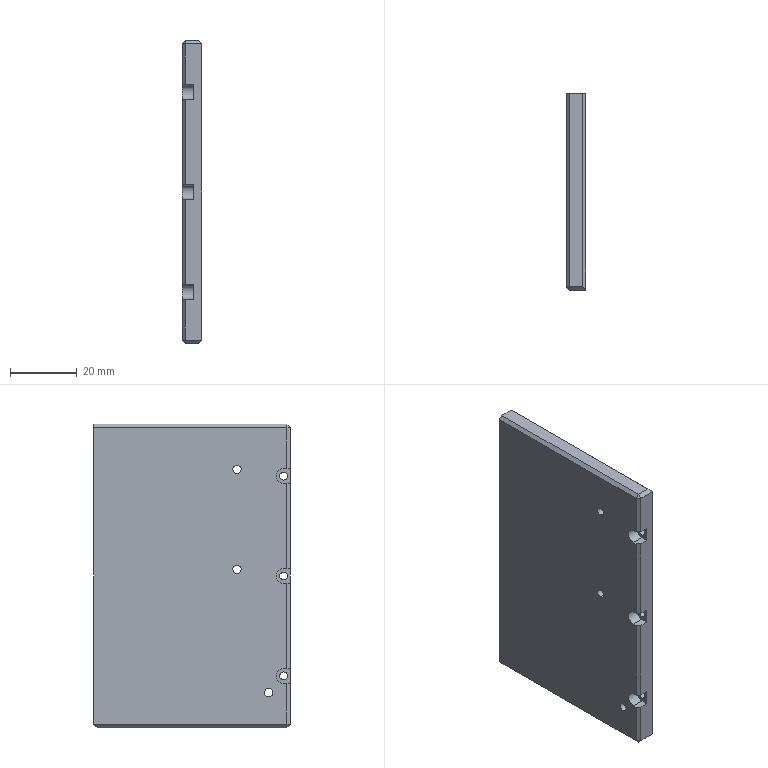CAM job | Mastercam | mm | 8 operations | part box 6 x 59 x 91
1. Contour (Ramp) | 7 - 4 平底刀
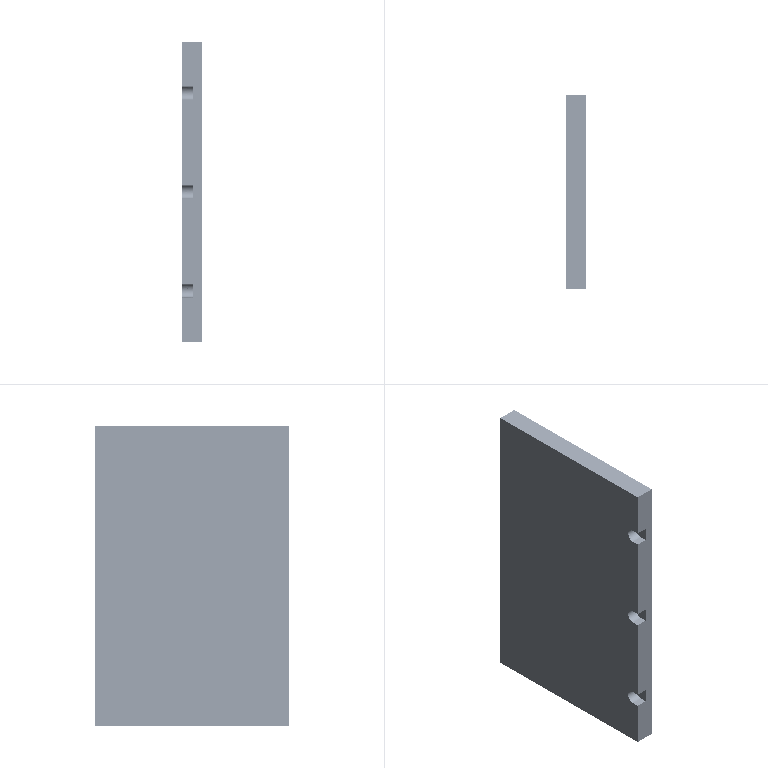2. Contour (2D) | 7 - 4 平底刀
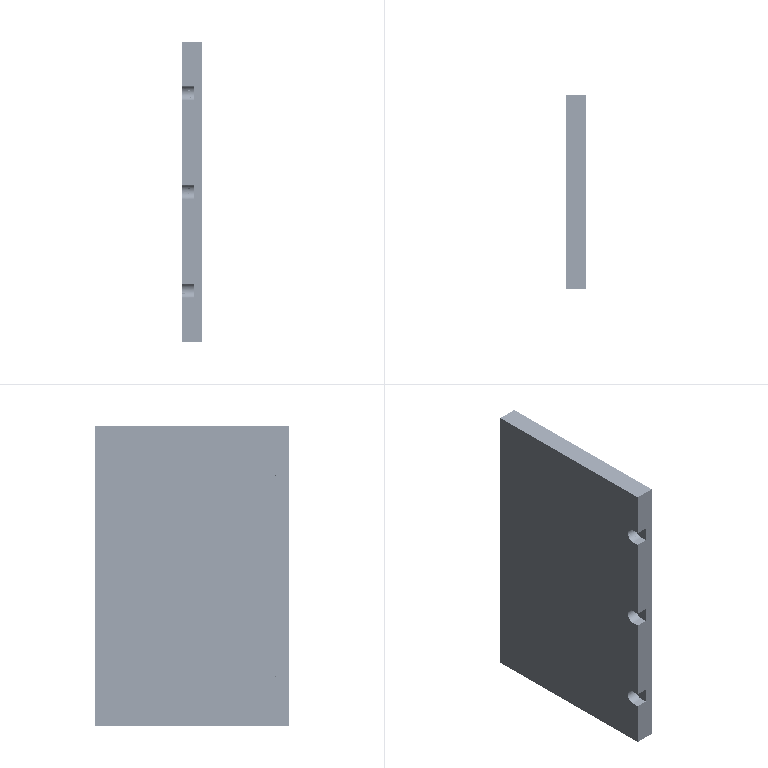3. Drill/Counterbore | 2 - 6定位倒角
4. Peck Drill | 12 - 2.5 钻头
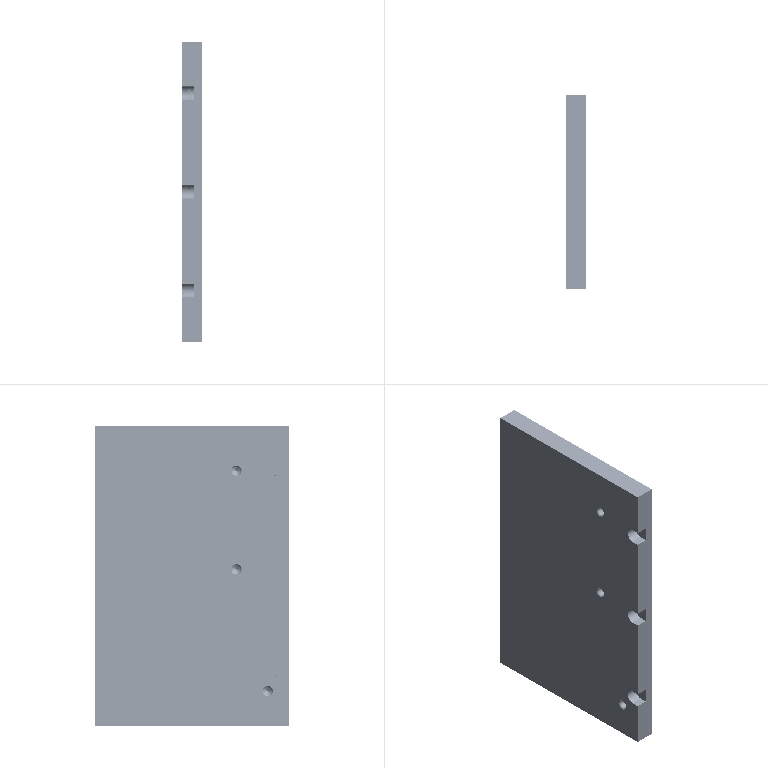5. Contour (2D chamfer) | 2 - 6定位倒角
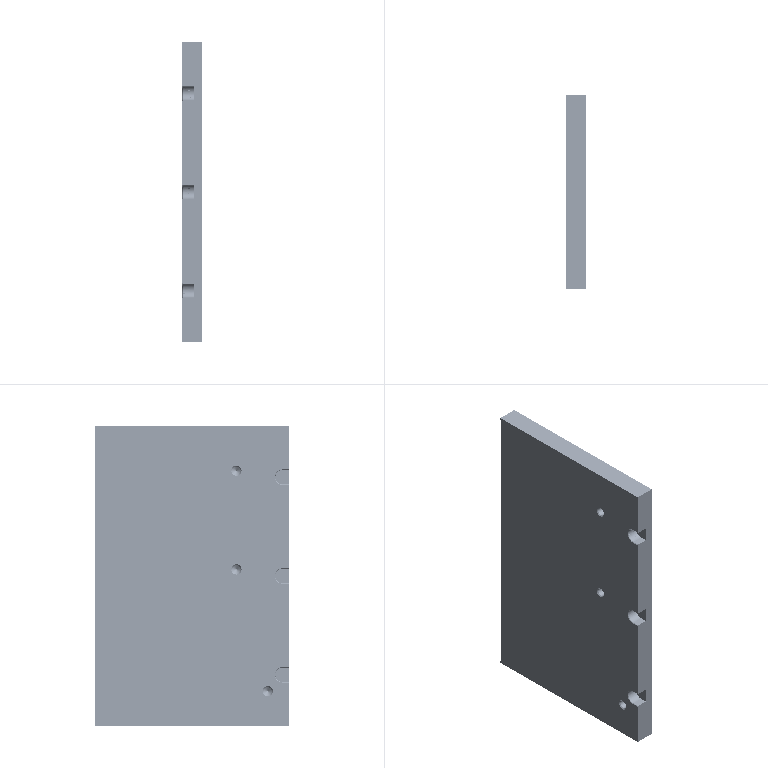6. Contour (2D chamfer) | 2 - 6定位倒角
7. Drill/Counterbore | 2 - 6定位倒角
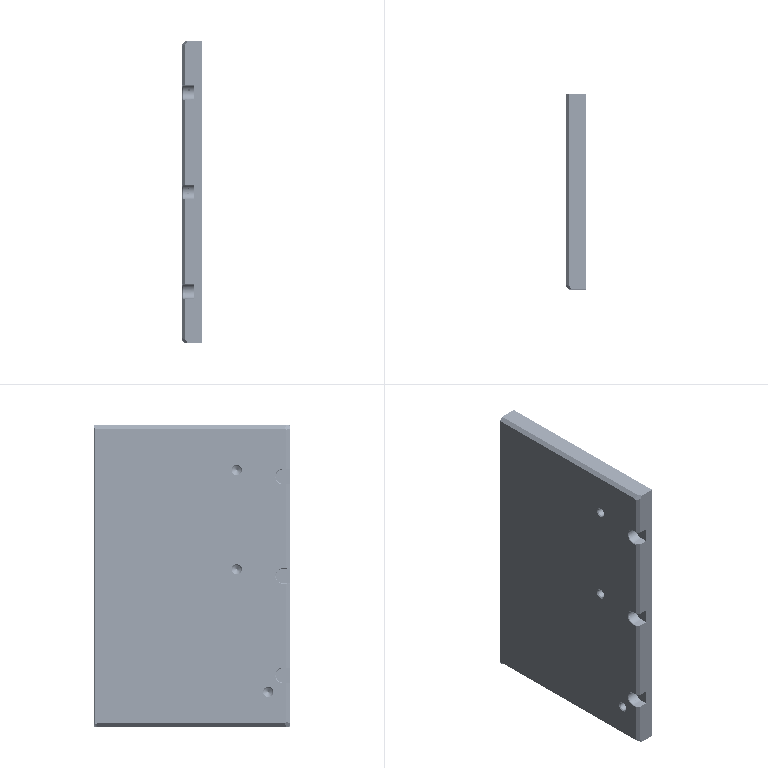8. Peck Drill | 12 - 2.5 钻头